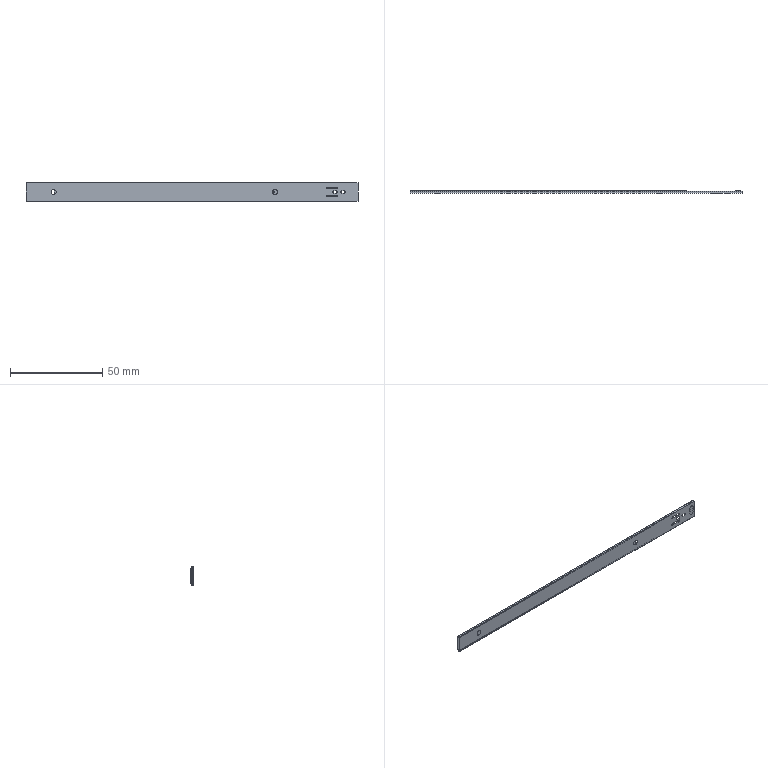Component | NX | SLIDE_RAIL_LARGE | 2 solids | 79 faces | volume 410 mm3 | plane 53 | cylinder 26 | commonest cylinder face diameters 1.5 x10 2.5 x4 1.2 x4 1 x4 3 x2 2.8 x2